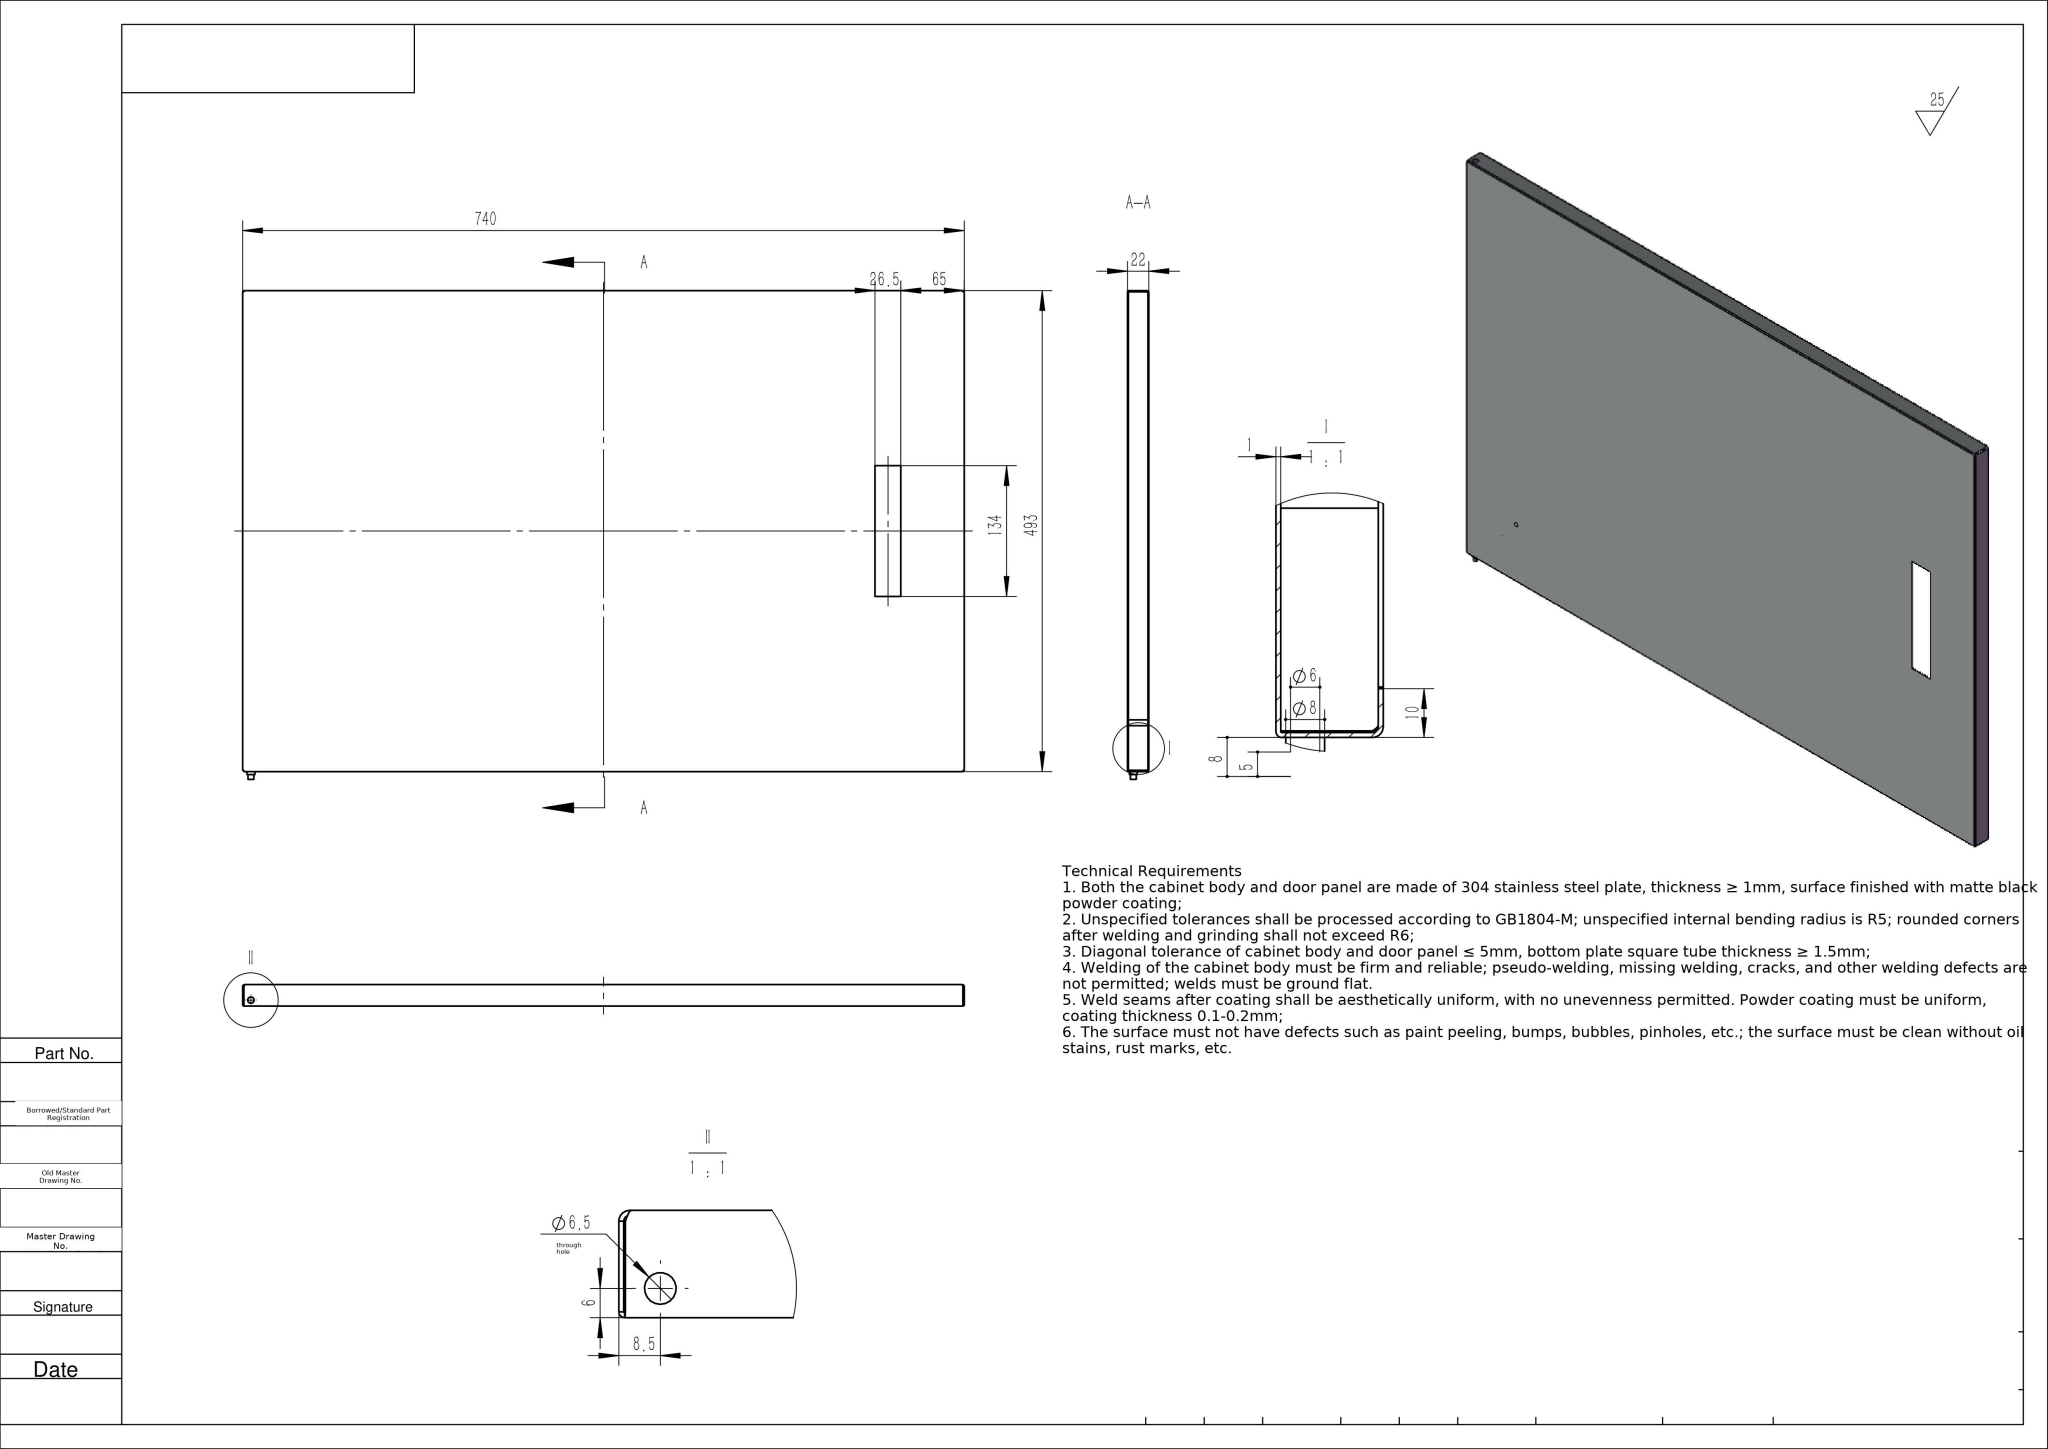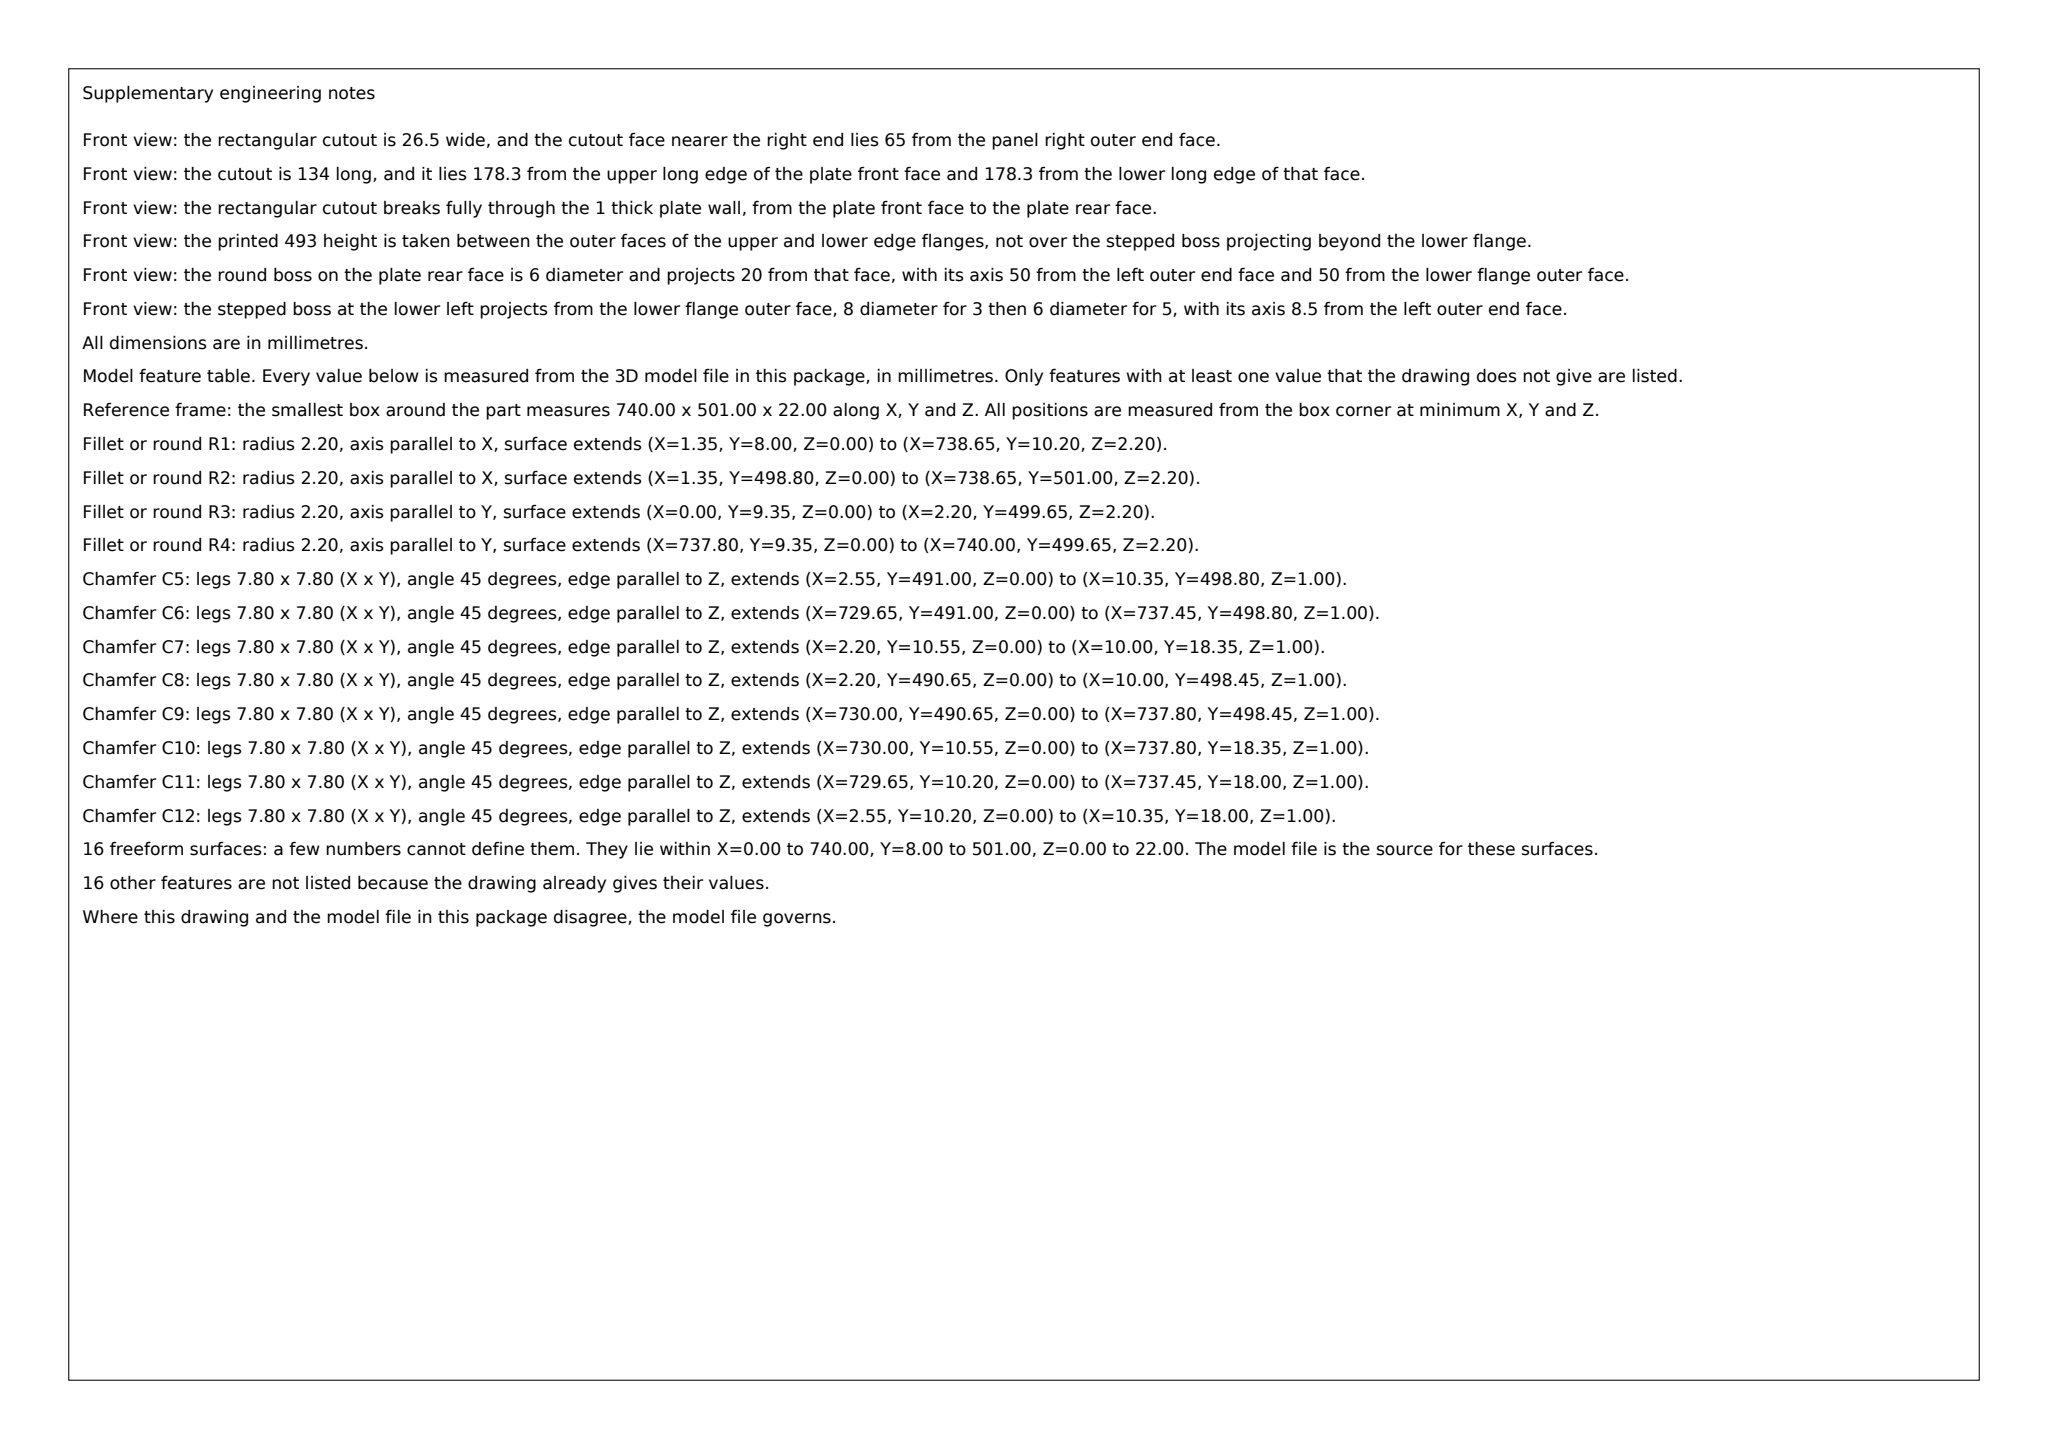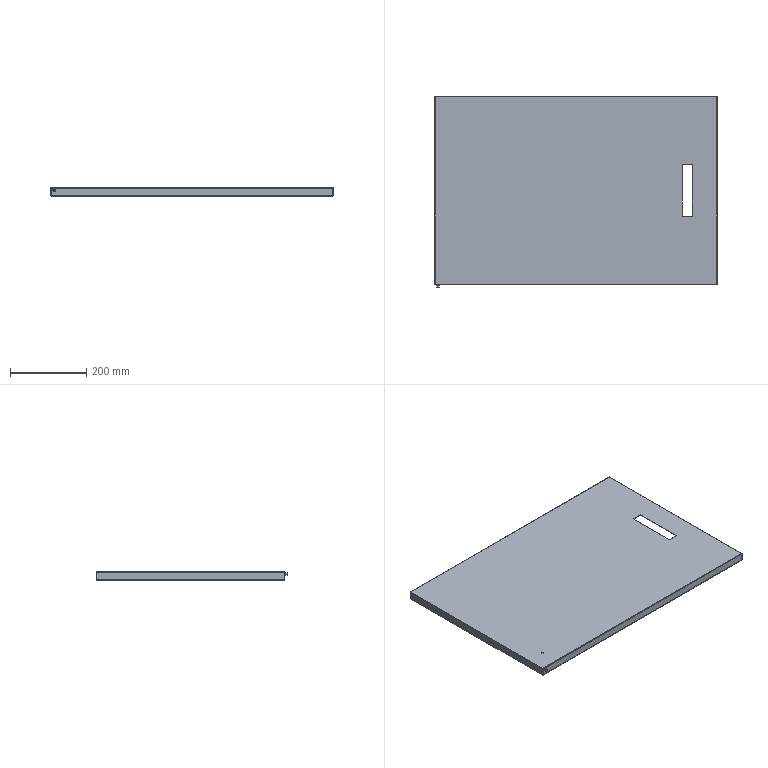Part | SolidWorks | mm | 1 solid | 85 faces | box 740 x 501 x 22 mm | volume 432882 mm3 | plane 45 | cylinder 24 | spline 16 | commonest cylinder face diameters 2.4 x8 6 x4 0.4 x4 4.4 x4 8 x2 6.5 x2
Drawing notes:
Overall plate height 501 (bbox Y); overall length 740, thickness 22. | from the solid: bbox_xyz = [740.02, 501.01, 22.02]
General tolerances per GB/T 1804-m (replaces unreadable note line 2). | from the solid: redacted garbled note 'GB1804-M' restored; no STEP dimension affected
Formed sheet-metal edges: inner bend radius R1.2, outer bend radius R2.2, typ all four folded edges (replaces unreadable R5/R6 callout). | from the solid: cylinders dia 2.4 (R1.2) and dia 4.4 (R2.2) running along X and Y edges, lengths 737.29/490.29
2X Ø6 hole, axis normal to face (Z), depth 20; one hole located X=50, Y=58 from lower-left corner of plate. | from the solid: cylinders [6.0,'z',[50.01,58.0],20.0], count 2
2X stepped hole in folded edge, axis parallel to Y, located X=8.5 and Z=16 from min corner, one at each Y end (TYP): Ø6.5 DP 1, then Ø8 DP 3, then Ø6 DP 5. | from the solid: cylinders [6.5,'y',[8.51,null,16.01],1.0,2], [8.0,'y',[8.51,null,16.01],3.0,2], [6.0,'y',[8.51,null,16.01],5.0,2]
Slot 26.5 wide x 134 high: slot centre 254.5 from bottom edge (4 above plate mid-height); slot sides at X=648.5 and X=675.0 from left edge. | from the solid: axis_planes y 187.5 and 321.5; axis_planes x 648.51 and 675.01
MATERIAL THICKNESS 1 (formed sheet): outer face Z=0 / inner face Z=1 on the main face, and X=0 to X=1 and X=739 to X=740 on the side walls. | from the solid: axis_planes z=0.01 & z=1.01; x=0.01 & 1.01; x=739.01 & 740.01 (1 mm offset pairs)
FOLDED EDGE SECTION (TYP 4 EDGES): flange depth 22 full plate thickness (Z=0 to Z=22); inside depth 20 (inner face of main skin Z=1 to inner face of return lip Z=21); return lip 1 thick, 9 wide from flange inner face - lip free edges at X=10.0, X=730.0, Y=18.0 and Y=491.0 from min corner. | from the solid: axis_planes z=21.01 & 22.01; x=10.01 & 730.01; y=18.0 & 491.0 with wall inner faces x=1.01/739.01, y=9.0/500.0
CORNER RELIEF AT ALL 4 FOLDED CORNERS: relief faces at X=1.36 and X=738.66, Y=9.35 and Y=499.65 from min corner, i.e. 0.35 clear of the flange inner faces (X=1.0/739.0, Y=9.0/500.0). | from the solid: axis_planes x=1.36 (2) & 738.66 (2); y=9.35 (2) & 499.65 (2) vs inner faces x=1.01/739.01, y=9.0/500.0
END LUG CARRYING THE STEPPED HOLE: lug projects 8 beyond the 493 plate edge - lug end face at Y=0, plate bottom edge at Y=8 from min corner (plate body Y=8 to Y=501). | from the solid: axis_planes y=0.0, y=8.0, y=501.0 (501-8 = 493 plate height); stepped-hole cylinders axis y at y-end
UNSPECIFIED RADII: R0.2 at the return-lip hem fold, TYP 4 EDGES - fold axes at Z=20.8 from outer face, running along X at Y=9.2 and Y=499.8 (737.6 long) and along Y at X=1.2 and X=738.8 (490.6 long), all from min corner of plate. | from the solid: cylinders dia 0.4: axis x at [y=9.2, z=20.81] and [y=499.8, z=20.81] length 737.6; axis y at [x=1.21, z=20.81] and [x=738.81, z=20.81] length 490.6